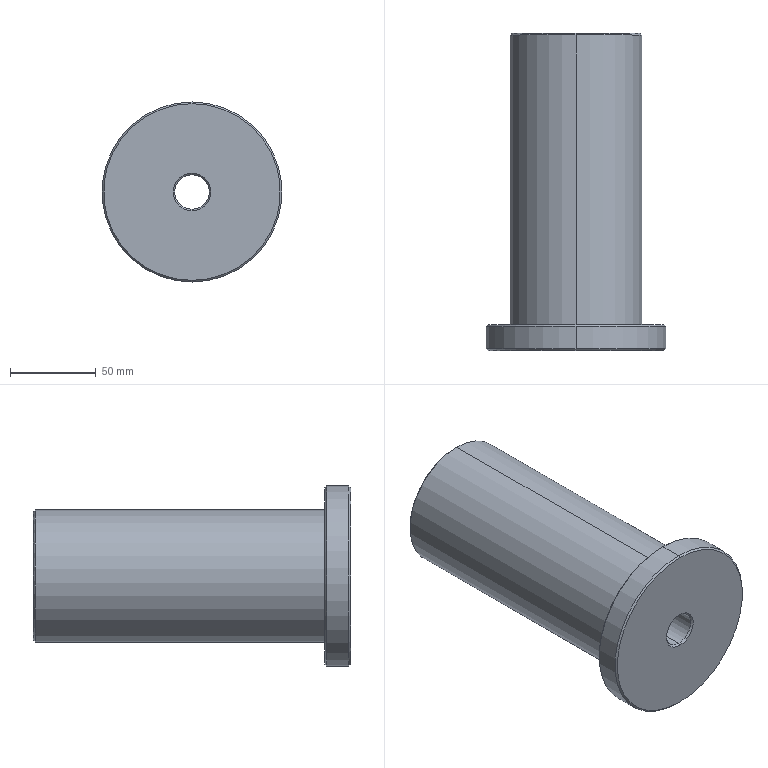Component | SolidWorks | 8TC-A15004-80-17A-2 | 1 solid | 19 faces | box 105 x 185 x 105 mm | volume 862880 mm3 | cone 10 | cylinder 6 | plane 3 | commonest cylinder face diameters 105 x2 20 x2 77 x2 | material Black POM
build123d program:
from build123d import *

# Parameters (mm, degrees)
CHAMFER1_SIZE = 1
CHAMFER2_SIZE = 1


with BuildPart() as part:
    # Sketch1 → Revolve1 (revolve)
    with BuildSketch(Plane(origin=(0, 0, 0), x_dir=(1, 0, 0), z_dir=(0, 1, 0)), mode=Mode.PRIVATE) as revolve1_sk:
        Polygon((185, 10), (185, 38.5), (15, 38.5), (15, 52.5), (0, 52.5), (0, 10), align=None)
    revolve(revolve1_sk.sketch.rotate(Axis((0, 0, 0), (1, 0, 0)), 180), axis=Axis((0, 0, 0), (1, 0, 0)))

    # Chamfer1
    chamfer1_edges = [part.edges().sort_by_distance(p)[0] for p in [
        (0, 0, -10),
        (185, 0, -10),
    ]]
    chamfer(chamfer1_edges, length=CHAMFER1_SIZE)

    # Chamfer2
    chamfer2_edges = [part.edges().sort_by_distance(p)[0] for p in [
        (15, 0, -52.5),
        (0, 0, -52.5),
        (185, 0, -38.5),
    ]]
    chamfer(chamfer2_edges, length=CHAMFER2_SIZE)


solid = part.part

# Placed as in the assembly
solid = solid.moved(Location((50, 22.5, 340), (0, 0, 90)))
STEP:
#1=COLOUR_RGB('',0.7922,0.8196,0.9333);
#2=FILL_AREA_STYLE_COLOUR('',#1);
#3=FILL_AREA_STYLE('',(#2));
#4=SURFACE_STYLE_FILL_AREA(#3);
#5=SURFACE_SIDE_STYLE('',(#4));
#6=SURFACE_STYLE_USAGE(.BOTH.,#5);
#7=PRESENTATION_STYLE_ASSIGNMENT((#6));
#8=CARTESIAN_POINT('',(1.969,8.169,11.909));
#9=VERTEX_POINT('',#8);
#10=CARTESIAN_POINT('',(1.969,8.169,14.862));
#11=VERTEX_POINT('',#10);
#12=CARTESIAN_POINT('',(1.969,8.169,13.386));
#13=DIRECTION('',(0.,1.,0.));
#14=DIRECTION('',(0.,0.,1.));
#15=AXIS2_PLACEMENT_3D('',#12,#13,#14);
#16=CIRCLE('',#15,1.476);
#17=EDGE_CURVE('',#9,#11,#16,.T.);
#18=ORIENTED_EDGE('',*,*,#17,.F.);
#19=CARTESIAN_POINT('',(1.969,8.13,11.87));
#20=VERTEX_POINT('',#19);
#21=CARTESIAN_POINT('',(1.969,8.13,11.87));
#22=DIRECTION('',(-0.,-0.7071,-0.7071));
#23=VECTOR('',#22,39.37);
#24=LINE('',#21,#23);
#25=EDGE_CURVE('',#9,#20,#24,.T.);
#26=ORIENTED_EDGE('',*,*,#25,.T.);
#27=CARTESIAN_POINT('',(1.969,8.13,14.902));
#28=VERTEX_POINT('',#27);
#29=CARTESIAN_POINT('',(1.969,8.13,13.386));
#30=DIRECTION('',(0.,-1.,0.));
#31=DIRECTION('',(0.,0.,1.));
#32=AXIS2_PLACEMENT_3D('',#29,#30,#31);
#33=CIRCLE('',#32,1.516);
#34=EDGE_CURVE('',#28,#20,#33,.T.);
#35=ORIENTED_EDGE('',*,*,#34,.F.);
#36=CARTESIAN_POINT('',(1.969,8.13,14.902));
#37=DIRECTION('',(0.,-0.7071,0.7071));
#38=VECTOR('',#37,39.37);
#39=LINE('',#36,#38);
#40=EDGE_CURVE('',#11,#28,#39,.T.);
#41=ORIENTED_EDGE('',*,*,#40,.F.);
#42=EDGE_LOOP('',(#18,#26,#35,#41));
#43=FACE_OUTER_BOUND('',#42,.T.);
#44=CARTESIAN_POINT('',(1.969,8.13,13.386));
#45=DIRECTION('',(0.,-1.,0.));
#46=DIRECTION('',(0.,0.,1.));
#47=AXIS2_PLACEMENT_3D('',#44,#45,#46);
#48=CONICAL_SURFACE('',#47,1.516,0.7854);
#49=ADVANCED_FACE('',(#43),#48,.T.);
#50=CARTESIAN_POINT('',(1.969,1.476,11.358));
#51=VERTEX_POINT('',#50);
#52=CARTESIAN_POINT('',(1.969,1.476,15.413));
#53=VERTEX_POINT('',#52);
#54=CARTESIAN_POINT('',(1.969,1.476,13.386));
#55=DIRECTION('',(0.,1.,0.));
#56=DIRECTION('',(0.,0.,1.));
#57=AXIS2_PLACEMENT_3D('',#54,#55,#56);
#58=CIRCLE('',#57,2.028);
#59=EDGE_CURVE('',#51,#53,#58,.T.);
#60=ORIENTED_EDGE('',*,*,#59,.F.);
#61=CARTESIAN_POINT('',(1.969,1.437,11.319));
#62=VERTEX_POINT('',#61);
#63=CARTESIAN_POINT('',(1.969,1.437,11.319));
#64=DIRECTION('',(-0.,-0.7071,-0.7071));
#65=VECTOR('',#64,39.37);
#66=LINE('',#63,#65);
#67=EDGE_CURVE('',#51,#62,#66,.T.);
#68=ORIENTED_EDGE('',*,*,#67,.T.);
#69=CARTESIAN_POINT('',(1.969,1.437,15.453));
#70=VERTEX_POINT('',#69);
#71=CARTESIAN_POINT('',(1.969,1.437,13.386));
#72=DIRECTION('',(0.,-1.,0.));
#73=DIRECTION('',(0.,0.,1.));
#74=AXIS2_PLACEMENT_3D('',#71,#72,#73);
#75=CIRCLE('',#74,2.067);
#76=EDGE_CURVE('',#70,#62,#75,.T.);
#77=ORIENTED_EDGE('',*,*,#76,.F.);
#78=CARTESIAN_POINT('',(1.969,1.437,15.453));
#79=DIRECTION('',(0.,-0.7071,0.7071));
#80=VECTOR('',#79,39.37);
#81=LINE('',#78,#80);
#82=EDGE_CURVE('',#53,#70,#81,.T.);
#83=ORIENTED_EDGE('',*,*,#82,.F.);
#84=EDGE_LOOP('',(#60,#68,#77,#83));
#85=FACE_OUTER_BOUND('',#84,.T.);
#86=CARTESIAN_POINT('',(1.969,1.437,13.386));
#87=DIRECTION('',(0.,-1.,0.));
#88=DIRECTION('',(0.,0.,1.));
#89=AXIS2_PLACEMENT_3D('',#86,#87,#88);
#90=CONICAL_SURFACE('',#89,2.067,0.7854);
#91=ADVANCED_FACE('',(#85),#90,.T.);
#92=CARTESIAN_POINT('',(1.969,0.8858,15.413));
#93=VERTEX_POINT('',#92);
#94=CARTESIAN_POINT('',(1.969,0.8858,11.358));
#95=VERTEX_POINT('',#94);
#96=CARTESIAN_POINT('',(1.969,0.8858,13.386));
#97=DIRECTION('',(0.,-1.,0.));
#98=DIRECTION('',(0.,0.,-1.));
#99=AXIS2_PLACEMENT_3D('',#96,#97,#98);
#100=CIRCLE('',#99,2.028);
#101=EDGE_CURVE('',#93,#95,#100,.T.);
#102=ORIENTED_EDGE('',*,*,#101,.F.);
#103=CARTESIAN_POINT('',(1.969,0.9252,15.453));
#104=VERTEX_POINT('',#103);
#105=CARTESIAN_POINT('',(1.969,0.8858,15.413));
#106=DIRECTION('',(-0.,0.7071,0.7071));
#107=VECTOR('',#106,39.37);
#108=LINE('',#105,#107);
#109=EDGE_CURVE('',#93,#104,#108,.T.);
#110=ORIENTED_EDGE('',*,*,#109,.T.);
#111=CARTESIAN_POINT('',(1.969,0.9252,11.319));
#112=VERTEX_POINT('',#111);
#113=CARTESIAN_POINT('',(1.969,0.9252,13.386));
#114=DIRECTION('',(0.,1.,0.));
#115=DIRECTION('',(0.,0.,-1.));
#116=AXIS2_PLACEMENT_3D('',#113,#114,#115);
#117=CIRCLE('',#116,2.067);
#118=EDGE_CURVE('',#112,#104,#117,.T.);
#119=ORIENTED_EDGE('',*,*,#118,.F.);
#120=CARTESIAN_POINT('',(1.969,0.8858,11.358));
#121=DIRECTION('',(0.,0.7071,-0.7071));
#122=VECTOR('',#121,39.37);
#123=LINE('',#120,#122);
#124=EDGE_CURVE('',#95,#112,#123,.T.);
#125=ORIENTED_EDGE('',*,*,#124,.F.);
#126=EDGE_LOOP('',(#102,#110,#119,#125));
#127=FACE_OUTER_BOUND('',#126,.T.);
#128=CARTESIAN_POINT('',(1.969,0.8858,13.386));
#129=DIRECTION('',(0.,1.,0.));
#130=DIRECTION('',(0.,0.,-1.));
#131=AXIS2_PLACEMENT_3D('',#128,#129,#130);
#132=CONICAL_SURFACE('',#131,2.028,0.7854);
#133=ADVANCED_FACE('',(#127),#132,.T.);
#134=CARTESIAN_POINT('',(1.969,0.9252,12.992));
#135=VERTEX_POINT('',#134);
#136=CARTESIAN_POINT('',(1.969,0.9252,13.78));
#137=VERTEX_POINT('',#136);
#138=CARTESIAN_POINT('',(1.969,0.9252,13.386));
#139=DIRECTION('',(0.,-1.,0.));
#140=DIRECTION('',(0.,0.,-1.));
#141=AXIS2_PLACEMENT_3D('',#138,#139,#140);
#142=CIRCLE('',#141,0.3937);
#143=EDGE_CURVE('',#135,#137,#142,.T.);
#144=ORIENTED_EDGE('',*,*,#143,.F.);
#145=CARTESIAN_POINT('',(1.969,0.8858,12.953));
#146=VERTEX_POINT('',#145);
#147=CARTESIAN_POINT('',(1.969,0.9252,12.992));
#148=DIRECTION('',(-0.,-0.7071,-0.7071));
#149=VECTOR('',#148,39.37);
#150=LINE('',#147,#149);
#151=EDGE_CURVE('',#135,#146,#150,.T.);
#152=ORIENTED_EDGE('',*,*,#151,.T.);
#153=CARTESIAN_POINT('',(1.969,0.8858,13.819));
#154=VERTEX_POINT('',#153);
#155=CARTESIAN_POINT('',(1.969,0.8858,13.386));
#156=DIRECTION('',(0.,1.,0.));
#157=DIRECTION('',(0.,0.,-1.));
#158=AXIS2_PLACEMENT_3D('',#155,#156,#157);
#159=CIRCLE('',#158,0.4331);
#160=EDGE_CURVE('',#154,#146,#159,.T.);
#161=ORIENTED_EDGE('',*,*,#160,.F.);
#162=CARTESIAN_POINT('',(1.969,0.9252,13.78));
#163=DIRECTION('',(0.,-0.7071,0.7071));
#164=VECTOR('',#163,39.37);
#165=LINE('',#162,#164);
#166=EDGE_CURVE('',#137,#154,#165,.T.);
#167=ORIENTED_EDGE('',*,*,#166,.F.);
#168=EDGE_LOOP('',(#144,#152,#161,#167));
#169=FACE_OUTER_BOUND('',#168,.T.);
#170=CARTESIAN_POINT('',(1.969,0.9252,13.386));
#171=DIRECTION('',(0.,-1.,0.));
#172=DIRECTION('',(0.,0.,1.));
#173=AXIS2_PLACEMENT_3D('',#170,#171,#172);
#174=CONICAL_SURFACE('',#173,0.3937,0.7854);
#175=ADVANCED_FACE('',(#169),#174,.F.);
#176=CARTESIAN_POINT('',(1.969,8.13,13.78));
#177=VERTEX_POINT('',#176);
#178=CARTESIAN_POINT('',(1.969,8.13,12.992));
#179=VERTEX_POINT('',#178);
#180=CARTESIAN_POINT('',(1.969,8.13,13.386));
#181=DIRECTION('',(0.,1.,0.));
#182=DIRECTION('',(0.,0.,1.));
#183=AXIS2_PLACEMENT_3D('',#180,#181,#182);
#184=CIRCLE('',#183,0.3937);
#185=EDGE_CURVE('',#177,#179,#184,.T.);
#186=ORIENTED_EDGE('',*,*,#185,.F.);
#187=CARTESIAN_POINT('',(1.969,8.169,13.819));
#188=VERTEX_POINT('',#187);
#189=CARTESIAN_POINT('',(1.969,8.169,13.819));
#190=DIRECTION('',(-0.,0.7071,0.7071));
#191=VECTOR('',#190,39.37);
#192=LINE('',#189,#191);
#193=EDGE_CURVE('',#177,#188,#192,.T.);
#194=ORIENTED_EDGE('',*,*,#193,.T.);
#195=CARTESIAN_POINT('',(1.969,8.169,12.953));
#196=VERTEX_POINT('',#195);
#197=CARTESIAN_POINT('',(1.969,8.169,13.386));
#198=DIRECTION('',(0.,-1.,0.));
#199=DIRECTION('',(0.,0.,1.));
#200=AXIS2_PLACEMENT_3D('',#197,#198,#199);
#201=CIRCLE('',#200,0.4331);
#202=EDGE_CURVE('',#196,#188,#201,.T.);
#203=ORIENTED_EDGE('',*,*,#202,.F.);
#204=CARTESIAN_POINT('',(1.969,8.169,12.953));
#205=DIRECTION('',(0.,0.7071,-0.7071));
#206=VECTOR('',#205,39.37);
#207=LINE('',#204,#206);
#208=EDGE_CURVE('',#179,#196,#207,.T.);
#209=ORIENTED_EDGE('',*,*,#208,.F.);
#210=EDGE_LOOP('',(#186,#194,#203,#209));
#211=FACE_OUTER_BOUND('',#210,.T.);
#212=CARTESIAN_POINT('',(1.969,8.169,13.386));
#213=DIRECTION('',(0.,1.,0.));
#214=DIRECTION('',(0.,0.,-1.));
#215=AXIS2_PLACEMENT_3D('',#212,#213,#214);
#216=CONICAL_SURFACE('',#215,0.4331,0.7854);
#217=ADVANCED_FACE('',(#211),#216,.F.);
#218=ORIENTED_EDGE('',*,*,#76,.T.);
#219=CARTESIAN_POINT('',(1.969,0.8858,11.319));
#220=DIRECTION('',(0.,-1.,0.));
#221=VECTOR('',#220,39.37);
#222=LINE('',#219,#221);
#223=EDGE_CURVE('',#62,#112,#222,.T.);
#224=ORIENTED_EDGE('',*,*,#223,.T.);
#225=ORIENTED_EDGE('',*,*,#118,.T.);
#226=CARTESIAN_POINT('',(1.969,0.8858,15.453));
#227=DIRECTION('',(0.,-1.,0.));
#228=VECTOR('',#227,39.37);
#229=LINE('',#226,#228);
#230=EDGE_CURVE('',#70,#104,#229,.T.);
#231=ORIENTED_EDGE('',*,*,#230,.F.);
#232=EDGE_LOOP('',(#218,#224,#225,#231));
#233=FACE_OUTER_BOUND('',#232,.T.);
#234=CARTESIAN_POINT('',(1.969,0.8858,13.386));
#235=DIRECTION('',(0.,-1.,0.));
#236=DIRECTION('',(0.,0.,1.));
#237=AXIS2_PLACEMENT_3D('',#234,#235,#236);
#238=CYLINDRICAL_SURFACE('',#237,2.067);
#239=ADVANCED_FACE('',(#233),#238,.T.);
#240=ORIENTED_EDGE('',*,*,#185,.T.);
#241=CARTESIAN_POINT('',(1.969,0.8858,12.992));
#242=DIRECTION('',(0.,-1.,0.));
#243=VECTOR('',#242,39.37);
#244=LINE('',#241,#243);
#245=EDGE_CURVE('',#179,#135,#244,.T.);
#246=ORIENTED_EDGE('',*,*,#245,.T.);
#247=ORIENTED_EDGE('',*,*,#143,.T.);
#248=CARTESIAN_POINT('',(1.969,0.8858,13.78));
#249=DIRECTION('',(0.,-1.,0.));
#250=VECTOR('',#249,39.37);
#251=LINE('',#248,#250);
#252=EDGE_CURVE('',#177,#137,#251,.T.);
#253=ORIENTED_EDGE('',*,*,#252,.F.);
#254=EDGE_LOOP('',(#240,#246,#247,#253));
#255=FACE_OUTER_BOUND('',#254,.T.);
#256=CARTESIAN_POINT('',(1.969,0.8858,13.386));
#257=DIRECTION('',(0.,-1.,0.));
#258=DIRECTION('',(0.,0.,1.));
#259=AXIS2_PLACEMENT_3D('',#256,#257,#258);
#260=CYLINDRICAL_SURFACE('',#259,0.3937);
#261=ADVANCED_FACE('',(#255),#260,.F.);
#262=ORIENTED_EDGE('',*,*,#34,.T.);
#263=CARTESIAN_POINT('',(1.969,1.476,11.87));
#264=VERTEX_POINT('',#263);
#265=CARTESIAN_POINT('',(1.969,0.8858,11.87));
#266=DIRECTION('',(0.,-1.,0.));
#267=VECTOR('',#266,39.37);
#268=LINE('',#265,#267);
#269=EDGE_CURVE('',#20,#264,#268,.T.);
#270=ORIENTED_EDGE('',*,*,#269,.T.);
#271=CARTESIAN_POINT('',(1.969,1.476,14.902));
#272=VERTEX_POINT('',#271);
#273=CARTESIAN_POINT('',(1.969,1.476,13.386));
#274=DIRECTION('',(0.,-1.,0.));
#275=DIRECTION('',(0.,0.,1.));
#276=AXIS2_PLACEMENT_3D('',#273,#274,#275);
#277=CIRCLE('',#276,1.516);
#278=EDGE_CURVE('',#272,#264,#277,.T.);
#279=ORIENTED_EDGE('',*,*,#278,.F.);
#280=CARTESIAN_POINT('',(1.969,0.8858,14.902));
#281=DIRECTION('',(0.,-1.,0.));
#282=VECTOR('',#281,39.37);
#283=LINE('',#280,#282);
#284=EDGE_CURVE('',#28,#272,#283,.T.);
#285=ORIENTED_EDGE('',*,*,#284,.F.);
#286=EDGE_LOOP('',(#262,#270,#279,#285));
#287=FACE_OUTER_BOUND('',#286,.T.);
#288=CARTESIAN_POINT('',(1.969,0.8858,13.386));
#289=DIRECTION('',(0.,-1.,0.));
#290=DIRECTION('',(0.,0.,1.));
#291=AXIS2_PLACEMENT_3D('',#288,#289,#290);
#292=CYLINDRICAL_SURFACE('',#291,1.516);
#293=ADVANCED_FACE('',(#287),#292,.T.);
#294=ORIENTED_EDGE('',*,*,#269,.F.);
#295=CARTESIAN_POINT('',(1.969,8.13,13.386));
#296=DIRECTION('',(0.,-1.,0.));
#297=DIRECTION('',(0.,0.,1.));
#298=AXIS2_PLACEMENT_3D('',#295,#296,#297);
#299=CIRCLE('',#298,1.516);
#300=EDGE_CURVE('',#20,#28,#299,.T.);
#301=ORIENTED_EDGE('',*,*,#300,.T.);
#302=ORIENTED_EDGE('',*,*,#284,.T.);
#303=CARTESIAN_POINT('',(1.969,1.476,13.386));
#304=DIRECTION('',(0.,-1.,0.));
#305=DIRECTION('',(0.,0.,1.));
#306=AXIS2_PLACEMENT_3D('',#303,#304,#305);
#307=CIRCLE('',#306,1.516);
#308=EDGE_CURVE('',#264,#272,#307,.T.);
#309=ORIENTED_EDGE('',*,*,#308,.F.);
#310=EDGE_LOOP('',(#294,#301,#302,#309));
#311=FACE_OUTER_BOUND('',#310,.T.);
#312=CARTESIAN_POINT('',(1.969,0.8858,13.386));
#313=DIRECTION('',(0.,-1.,0.));
#314=DIRECTION('',(0.,0.,1.));
#315=AXIS2_PLACEMENT_3D('',#312,#313,#314);
#316=CYLINDRICAL_SURFACE('',#315,1.516);
#317=ADVANCED_FACE('',(#311),#316,.T.);
#318=CARTESIAN_POINT('',(1.969,8.169,13.386));
#319=DIRECTION('',(0.,1.,0.));
#320=DIRECTION('',(0.,0.,1.));
#321=AXIS2_PLACEMENT_3D('',#318,#319,#320);
#322=CIRCLE('',#321,1.476);
#323=EDGE_CURVE('',#11,#9,#322,.T.);
#324=ORIENTED_EDGE('',*,*,#323,.T.);
#325=ORIENTED_EDGE('',*,*,#17,.T.);
#326=EDGE_LOOP('',(#324,#325));
#327=FACE_OUTER_BOUND('',#326,.T.);
#328=ORIENTED_EDGE('',*,*,#202,.T.);
#329=CARTESIAN_POINT('',(1.969,8.169,13.386));
#330=DIRECTION('',(0.,-1.,0.));
#331=DIRECTION('',(0.,0.,1.));
#332=AXIS2_PLACEMENT_3D('',#329,#330,#331);
#333=CIRCLE('',#332,0.4331);
#334=EDGE_CURVE('',#188,#196,#333,.T.);
#335=ORIENTED_EDGE('',*,*,#334,.T.);
#336=EDGE_LOOP('',(#328,#335));
#337=FACE_BOUND('',#336,.T.);
#338=CARTESIAN_POINT('',(1.969,8.169,12.992));
#339=DIRECTION('',(0.,-1.,0.));
#340=DIRECTION('',(0.,0.,1.));
#341=AXIS2_PLACEMENT_3D('',#338,#339,#340);
#342=PLANE('',#341);
#343=ADVANCED_FACE('',(#327,#337),#342,.F.);
#344=ORIENTED_EDGE('',*,*,#245,.F.);
#345=CARTESIAN_POINT('',(1.969,8.13,13.386));
#346=DIRECTION('',(0.,1.,0.));
#347=DIRECTION('',(0.,0.,1.));
#348=AXIS2_PLACEMENT_3D('',#345,#346,#347);
#349=CIRCLE('',#348,0.3937);
#350=EDGE_CURVE('',#179,#177,#349,.T.);
#351=ORIENTED_EDGE('',*,*,#350,.T.);
#352=ORIENTED_EDGE('',*,*,#252,.T.);
#353=CARTESIAN_POINT('',(1.969,0.9252,13.386));
#354=DIRECTION('',(0.,-1.,0.));
#355=DIRECTION('',(0.,0.,-1.));
#356=AXIS2_PLACEMENT_3D('',#353,#354,#355);
#357=CIRCLE('',#356,0.3937);
#358=EDGE_CURVE('',#137,#135,#357,.T.);
#359=ORIENTED_EDGE('',*,*,#358,.T.);
#360=EDGE_LOOP('',(#344,#351,#352,#359));
#361=FACE_OUTER_BOUND('',#360,.T.);
#362=CARTESIAN_POINT('',(1.969,0.8858,13.386));
#363=DIRECTION('',(0.,-1.,0.));
#364=DIRECTION('',(0.,0.,1.));
#365=AXIS2_PLACEMENT_3D('',#362,#363,#364);
#366=CYLINDRICAL_SURFACE('',#365,0.3937);
#367=ADVANCED_FACE('',(#361),#366,.F.);
#368=CARTESIAN_POINT('',(1.969,0.8858,13.386));
#369=DIRECTION('',(0.,-1.,0.));
#370=DIRECTION('',(0.,0.,-1.));
#371=AXIS2_PLACEMENT_3D('',#368,#369,#370);
#372=CIRCLE('',#371,2.028);
#373=EDGE_CURVE('',#95,#93,#372,.T.);
#374=ORIENTED_EDGE('',*,*,#373,.T.);
#375=ORIENTED_EDGE('',*,*,#101,.T.);
#376=EDGE_LOOP('',(#374,#375));
#377=FACE_OUTER_BOUND('',#376,.T.);
#378=ORIENTED_EDGE('',*,*,#160,.T.);
#379=CARTESIAN_POINT('',(1.969,0.8858,13.386));
#380=DIRECTION('',(0.,1.,0.));
#381=DIRECTION('',(0.,0.,-1.));
#382=AXIS2_PLACEMENT_3D('',#379,#380,#381);
#383=CIRCLE('',#382,0.4331);
#384=EDGE_CURVE('',#146,#154,#383,.T.);
#385=ORIENTED_EDGE('',*,*,#384,.T.);
#386=EDGE_LOOP('',(#378,#385));
#387=FACE_BOUND('',#386,.T.);
#388=CARTESIAN_POINT('',(1.969,0.8858,11.319));
#389=DIRECTION('',(0.,1.,0.));
#390=DIRECTION('',(0.,0.,-1.));
#391=AXIS2_PLACEMENT_3D('',#388,#389,#390);
#392=PLANE('',#391);
#393=ADVANCED_FACE('',(#377,#387),#392,.F.);
#394=ORIENTED_EDGE('',*,*,#223,.F.);
#395=CARTESIAN_POINT('',(1.969,1.437,13.386));
#396=DIRECTION('',(0.,-1.,0.));
#397=DIRECTION('',(0.,0.,1.));
#398=AXIS2_PLACEMENT_3D('',#395,#396,#397);
#399=CIRCLE('',#398,2.067);
#400=EDGE_CURVE('',#62,#70,#399,.T.);
#401=ORIENTED_EDGE('',*,*,#400,.T.);
#402=ORIENTED_EDGE('',*,*,#230,.T.);
#403=CARTESIAN_POINT('',(1.969,0.9252,13.386));
#404=DIRECTION('',(0.,1.,0.));
#405=DIRECTION('',(0.,0.,-1.));
#406=AXIS2_PLACEMENT_3D('',#403,#404,#405);
#407=CIRCLE('',#406,2.067);
#408=EDGE_CURVE('',#104,#112,#407,.T.);
#409=ORIENTED_EDGE('',*,*,#408,.T.);
#410=EDGE_LOOP('',(#394,#401,#402,#409));
#411=FACE_OUTER_BOUND('',#410,.T.);
#412=CARTESIAN_POINT('',(1.969,0.8858,13.386));
#413=DIRECTION('',(0.,-1.,0.));
#414=DIRECTION('',(0.,0.,1.));
#415=AXIS2_PLACEMENT_3D('',#412,#413,#414);
#416=CYLINDRICAL_SURFACE('',#415,2.067);
#417=ADVANCED_FACE('',(#411),#416,.T.);
#418=CARTESIAN_POINT('',(1.969,1.476,13.386));
#419=DIRECTION('',(0.,1.,0.));
#420=DIRECTION('',(0.,0.,1.));
#421=AXIS2_PLACEMENT_3D('',#418,#419,#420);
#422=CIRCLE('',#421,2.028);
#423=EDGE_CURVE('',#53,#51,#422,.T.);
#424=ORIENTED_EDGE('',*,*,#423,.T.);
#425=ORIENTED_EDGE('',*,*,#59,.T.);
#426=EDGE_LOOP('',(#424,#425));
#427=FACE_OUTER_BOUND('',#426,.T.);
#428=ORIENTED_EDGE('',*,*,#278,.T.);
#429=ORIENTED_EDGE('',*,*,#308,.T.);
#430=EDGE_LOOP('',(#428,#429));
#431=FACE_BOUND('',#430,.T.);
#432=CARTESIAN_POINT('',(1.969,1.476,11.87));
#433=DIRECTION('',(0.,-1.,0.));
#434=DIRECTION('',(0.,0.,1.));
#435=AXIS2_PLACEMENT_3D('',#432,#433,#434);
#436=PLANE('',#435);
#437=ADVANCED_FACE('',(#427,#431),#436,.F.);
#438=ORIENTED_EDGE('',*,*,#193,.F.);
#439=ORIENTED_EDGE('',*,*,#350,.F.);
#440=ORIENTED_EDGE('',*,*,#208,.T.);
#441=ORIENTED_EDGE('',*,*,#334,.F.);
#442=EDGE_LOOP('',(#438,#439,#440,#441));
#443=FACE_OUTER_BOUND('',#442,.T.);
#444=CARTESIAN_POINT('',(1.969,8.169,13.386));
#445=DIRECTION('',(0.,1.,0.));
#446=DIRECTION('',(0.,0.,-1.));
#447=AXIS2_PLACEMENT_3D('',#444,#445,#446);
#448=CONICAL_SURFACE('',#447,0.4331,0.7854);
#449=ADVANCED_FACE('',(#443),#448,.F.);
#450=ORIENTED_EDGE('',*,*,#151,.F.);
#451=ORIENTED_EDGE('',*,*,#358,.F.);
#452=ORIENTED_EDGE('',*,*,#166,.T.);
#453=ORIENTED_EDGE('',*,*,#384,.F.);
#454=EDGE_LOOP('',(#450,#451,#452,#453));
#455=FACE_OUTER_BOUND('',#454,.T.);
#456=CARTESIAN_POINT('',(1.969,0.9252,13.386));
#457=DIRECTION('',(0.,-1.,0.));
#458=DIRECTION('',(0.,0.,1.));
#459=AXIS2_PLACEMENT_3D('',#456,#457,#458);
#460=CONICAL_SURFACE('',#459,0.3937,0.7854);
#461=ADVANCED_FACE('',(#455),#460,.F.);
#462=ORIENTED_EDGE('',*,*,#109,.F.);
#463=ORIENTED_EDGE('',*,*,#373,.F.);
#464=ORIENTED_EDGE('',*,*,#124,.T.);
#465=ORIENTED_EDGE('',*,*,#408,.F.);
#466=EDGE_LOOP('',(#462,#463,#464,#465));
#467=FACE_OUTER_BOUND('',#466,.T.);
#468=CARTESIAN_POINT('',(1.969,0.8858,13.386));
#469=DIRECTION('',(0.,1.,0.));
#470=DIRECTION('',(0.,0.,-1.));
#471=AXIS2_PLACEMENT_3D('',#468,#469,#470);
#472=CONICAL_SURFACE('',#471,2.028,0.7854);
#473=ADVANCED_FACE('',(#467),#472,.T.);
#474=ORIENTED_EDGE('',*,*,#67,.F.);
#475=ORIENTED_EDGE('',*,*,#423,.F.);
#476=ORIENTED_EDGE('',*,*,#82,.T.);
#477=ORIENTED_EDGE('',*,*,#400,.F.);
#478=EDGE_LOOP('',(#474,#475,#476,#477));
#479=FACE_OUTER_BOUND('',#478,.T.);
#480=CARTESIAN_POINT('',(1.969,1.437,13.386));
#481=DIRECTION('',(0.,-1.,0.));
#482=DIRECTION('',(0.,0.,1.));
#483=AXIS2_PLACEMENT_3D('',#480,#481,#482);
#484=CONICAL_SURFACE('',#483,2.067,0.7854);
#485=ADVANCED_FACE('',(#479),#484,.T.);
#486=ORIENTED_EDGE('',*,*,#25,.F.);
#487=ORIENTED_EDGE('',*,*,#323,.F.);
#488=ORIENTED_EDGE('',*,*,#40,.T.);
#489=ORIENTED_EDGE('',*,*,#300,.F.);
#490=EDGE_LOOP('',(#486,#487,#488,#489));
#491=FACE_OUTER_BOUND('',#490,.T.);
#492=CARTESIAN_POINT('',(1.969,8.13,13.386));
#493=DIRECTION('',(0.,-1.,0.));
#494=DIRECTION('',(0.,0.,1.));
#495=AXIS2_PLACEMENT_3D('',#492,#493,#494);
#496=CONICAL_SURFACE('',#495,1.516,0.7854);
#497=ADVANCED_FACE('',(#491),#496,.T.);
#498=CLOSED_SHELL('',(#49,#91,#133,#175,#217,#239,#261,#293,#317,#343,#367,#393,#417,#437,#449,#461,#473,#485,#497));
#499=MANIFOLD_SOLID_BREP('',#498);
#500=STYLED_ITEM('',(#7),#499);
#501=(LENGTH_UNIT()NAMED_UNIT(*)SI_UNIT($,.METRE.));
#502=LENGTH_MEASURE_WITH_UNIT(LENGTH_MEASURE(0.0254),#501);
#503=DIMENSIONAL_EXPONENTS(1.,0.,0.,0.,0.,0.,0.);
#504=(CONVERSION_BASED_UNIT('',#502)LENGTH_UNIT()NAMED_UNIT(#503));
#505=UNCERTAINTY_MEASURE_WITH_UNIT(LENGTH_MEASURE(0.00001),#504,'','');
#506=(NAMED_UNIT(*)PLANE_ANGLE_UNIT()SI_UNIT($,.RADIAN.));
#507=(NAMED_UNIT(*)SI_UNIT($,.STERADIAN.)SOLID_ANGLE_UNIT());
#508=(GEOMETRIC_REPRESENTATION_CONTEXT(3)GLOBAL_UNCERTAINTY_ASSIGNED_CONTEXT((#505))GLOBAL_UNIT_ASSIGNED_CONTEXT((#504,#506,#507))REPRESENTATION_CONTEXT('',''));
#509=MECHANICAL_DESIGN_GEOMETRIC_PRESENTATION_REPRESENTATION('',(#500),#508);
#510=CARTESIAN_POINT('',(0.,0.,0.));
#511=DIRECTION('',(0.,0.,1.));
#512=DIRECTION('',(1.,0.,0.));
#513=AXIS2_PLACEMENT_3D('',#510,#511,#512);
#514=(LENGTH_UNIT()NAMED_UNIT(*)SI_UNIT($,.METRE.));
#515=LENGTH_MEASURE_WITH_UNIT(LENGTH_MEASURE(0.0254),#514);
#516=DIMENSIONAL_EXPONENTS(1.,0.,0.,0.,0.,0.,0.);
#517=(CONVERSION_BASED_UNIT('',#515)LENGTH_UNIT()NAMED_UNIT(#516));
#518=UNCERTAINTY_MEASURE_WITH_UNIT(LENGTH_MEASURE(0.00001),#517,'','');
#519=(NAMED_UNIT(*)PLANE_ANGLE_UNIT()SI_UNIT($,.RADIAN.));
#520=(NAMED_UNIT(*)SI_UNIT($,.STERADIAN.)SOLID_ANGLE_UNIT());
#521=(GEOMETRIC_REPRESENTATION_CONTEXT(3)GLOBAL_UNCERTAINTY_ASSIGNED_CONTEXT((#518))GLOBAL_UNIT_ASSIGNED_CONTEXT((#517,#519,#520))REPRESENTATION_CONTEXT('',''));
#522=ADVANCED_BREP_SHAPE_REPRESENTATION('',(#499,#513),#521);
#523=PRESENTATION_LAYER_ASSIGNMENT('','',(#500));